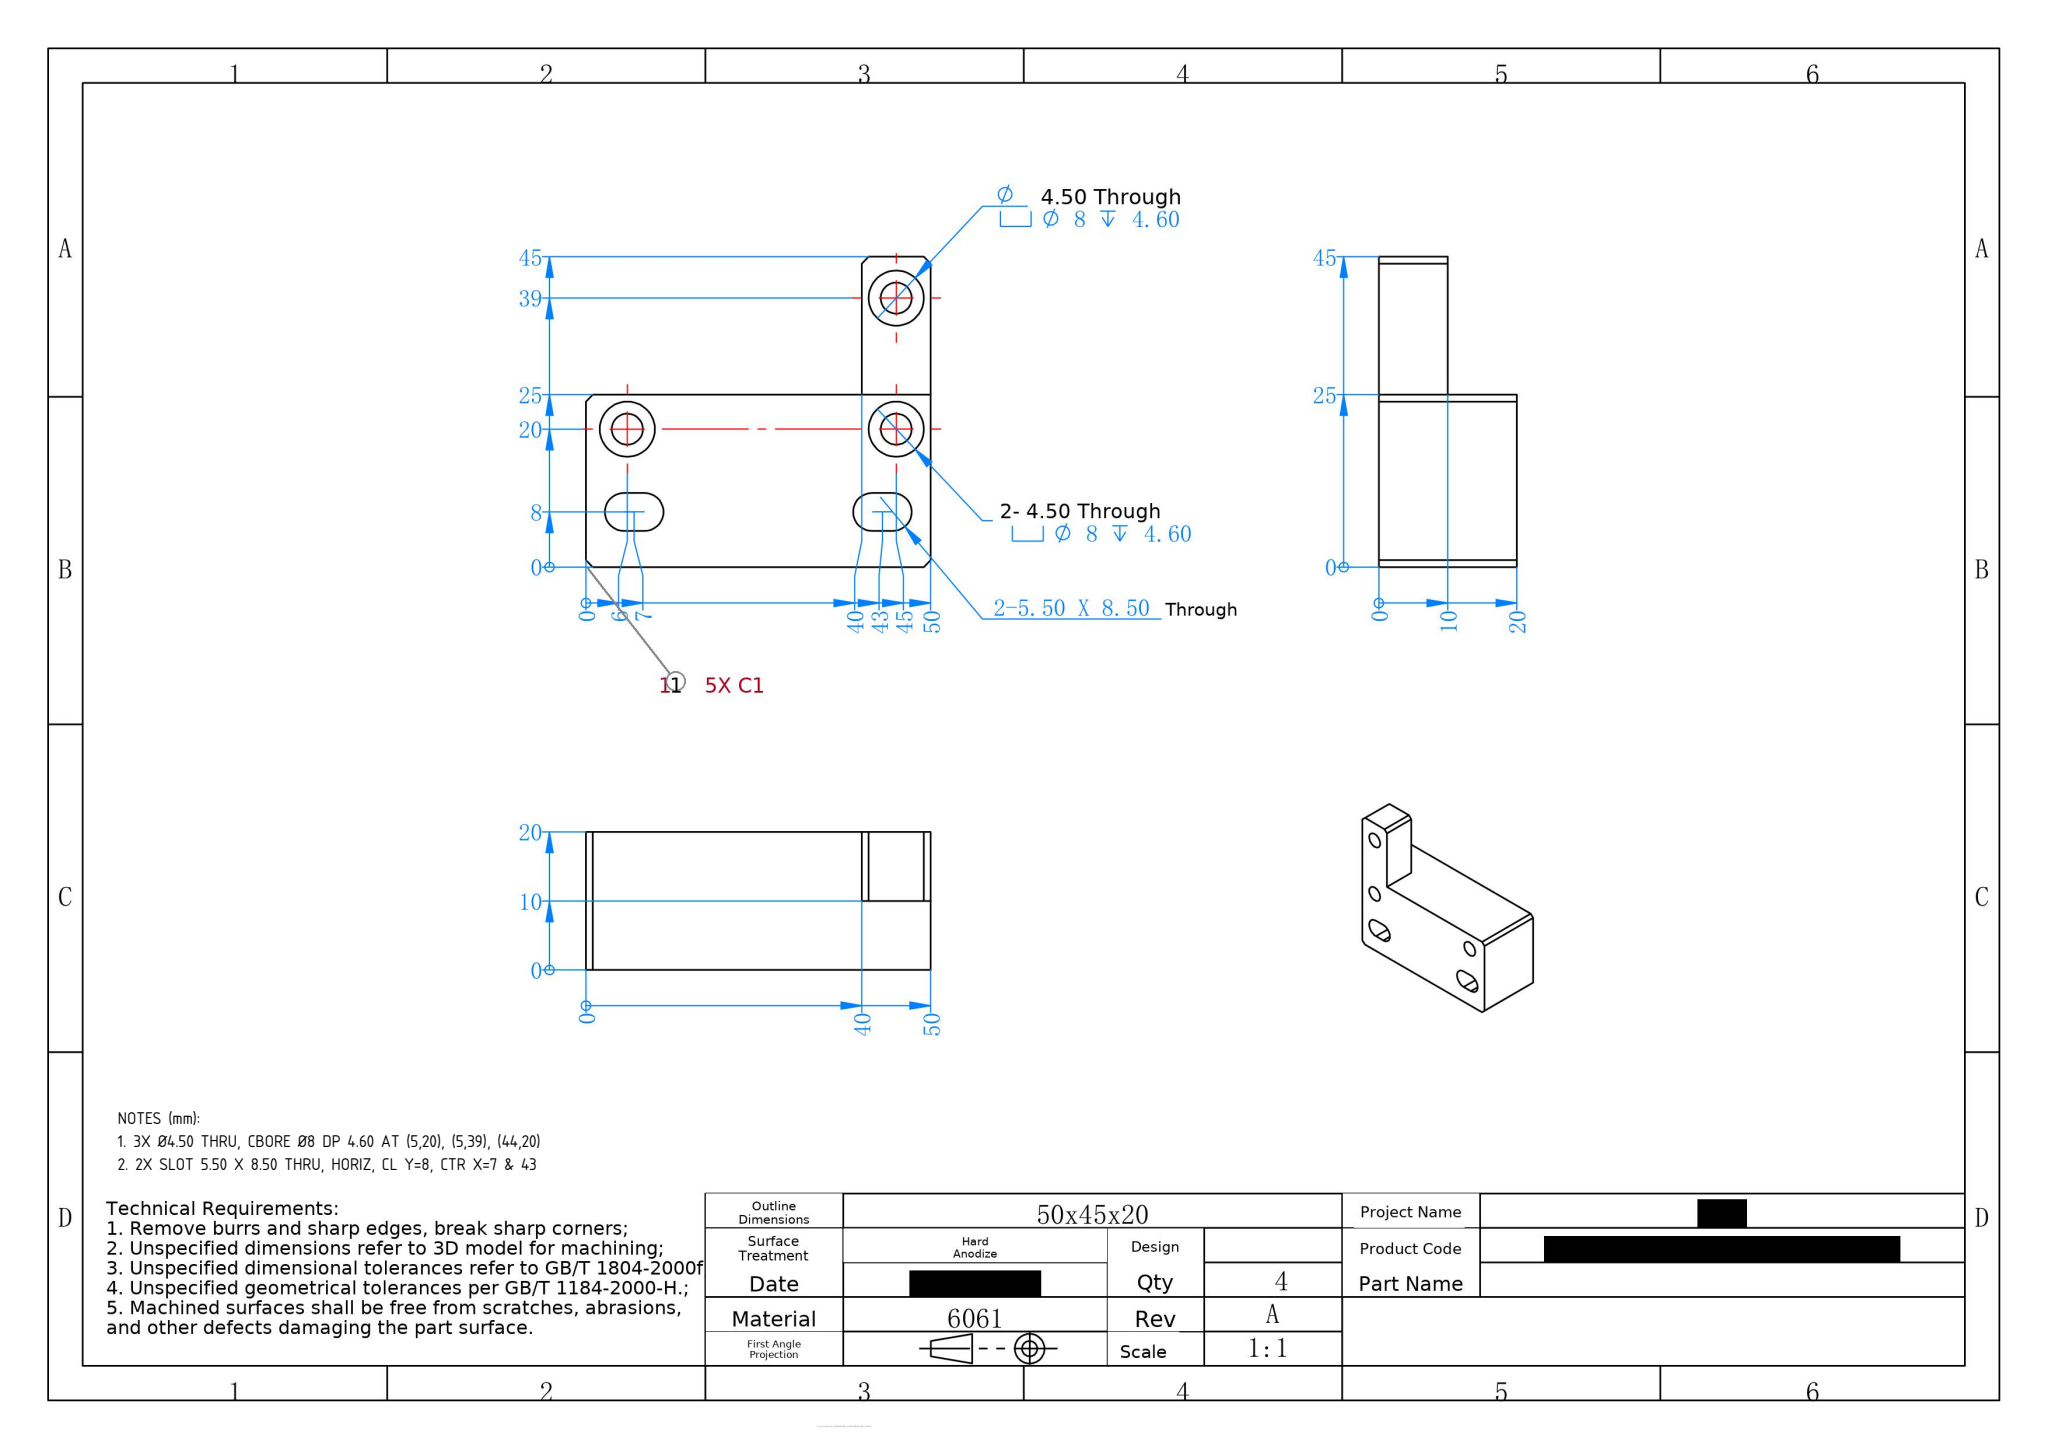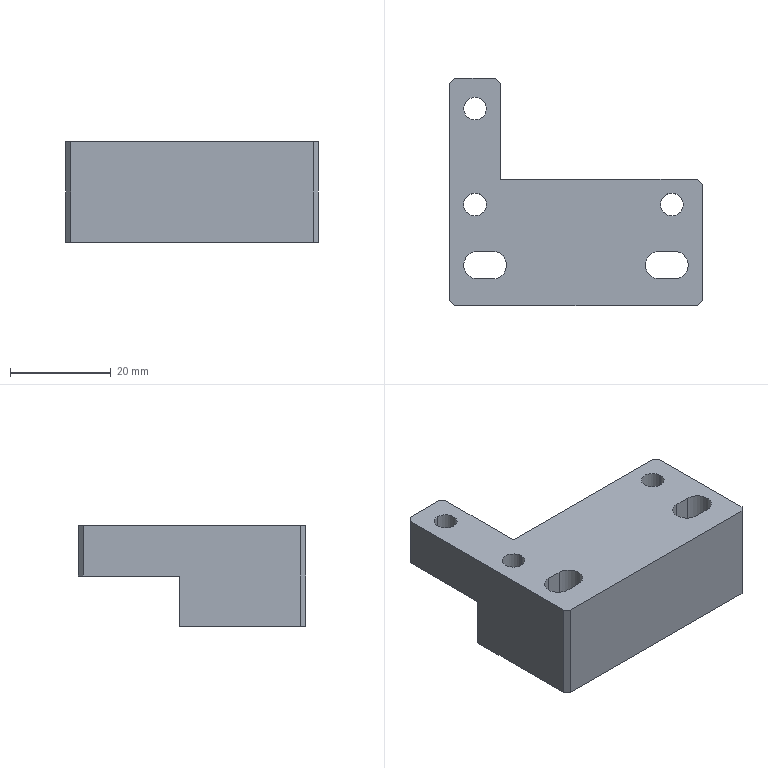Part | SolidWorks | mm | 1 solid | 39 faces | box 50 x 45 x 20 mm | volume 24080 mm3 | plane 21 | cylinder 18 | commonest cylinder face diameters 5.5 x6 8 x6 4.5 x6
Drawing notes:
3X Ø4.50 THRU, CBORE Ø8 DP 4.60 AT (5,20), (5,39), (44,20) | from the solid: cyl Ø4.5 z at (5,20),(5,39),(44,20); Ø8 CBORE 4.6 deep at same centres
2X SLOT 5.50 X 8.50 THRU, HORIZ, CL Y=8, CTR X=7 & 43 | from the solid: Ø5.5 thru end cyls at (5.5,8)&(8.5,8) and (41.5,8)&(44.5,8), len 20 = thru